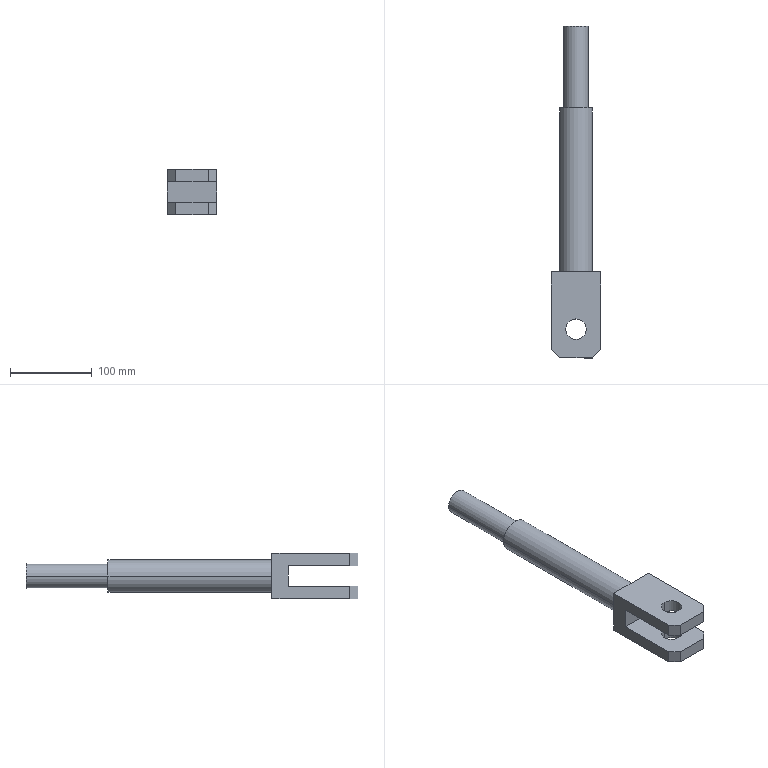Component | SolidWorks | Left-handTieRod1-1 | 1 solid | 24 faces | box 60 x 405 x 55 mm | volume 523287 mm3 | plane 16 | cylinder 8 | commonest cylinder face diameters 25 x4 30 x2 40 x2 | material N/A
build123d program:
from build123d import *

# Parameters (mm, degrees)
BOSS_EXTRUDE1_DEPTH = 30
SKETCH2_R           = 12.5
CUT_EXTRUDE1_DEPTH  = 60
CHAMFER1_SIZE       = 10
SKETCH3_R           = 20
BOSS_EXTRUDE2_DEPTH = 300
SKETCH4_OUTSIDE_W   = 144.62
SKETCH4_OUTSIDE_H   = 139.62
SKETCH4_OUTSIDE_R   = 15
CUT_EXTRUDE2_DEPTH  = 100


with BuildPart() as part:
    # Sketch1 → Boss-Extrude1 (new, symmetric)
    with BuildSketch(Plane(origin=(0, 0, 0), x_dir=(0, 0, -1), z_dir=(1, 0, 0))):
        Polygon((52.5, 12.5), (-32.5, 12.5), (-32.5, -12.5), (52.5, -12.5), (52.5, -27.5), (-52.5, -27.5), (-52.5, 27.5), (52.5, 27.5), align=None)
    extrude(amount=BOSS_EXTRUDE1_DEPTH, both=True)

    # Sketch2 → Cut-Extrude1 (cut)
    with BuildSketch(Plane.XZ.offset(27.5)):
        with Locations(Location((0, -17.5, 0), (0, 0, 270))):
            Circle(SKETCH2_R)
    extrude(amount=-CUT_EXTRUDE1_DEPTH, mode=Mode.SUBTRACT)

    # Chamfer1
    chamfer1_edges = [part.edges().sort_by_distance(p)[0] for p in [
        (-30, 20, -52.5),
        (30, -20, -52.5),
        (30, 20, -52.5),
        (-30, -20, -52.5),
    ]]
    chamfer(chamfer1_edges, length=CHAMFER1_SIZE)

    # Sketch3 → Boss-Extrude2 (add)
    with BuildSketch(Plane.XY.offset(52.5)):
        Circle(SKETCH3_R)
    extrude(amount=BOSS_EXTRUDE2_DEPTH)

    # Sketch4 outside → Cut-Extrude2 (cut)
    with BuildSketch(Plane.XY.offset(352.5)):
        Rectangle(SKETCH4_OUTSIDE_W, SKETCH4_OUTSIDE_H)
        Circle(SKETCH4_OUTSIDE_R, mode=Mode.SUBTRACT)
    extrude(amount=-CUT_EXTRUDE2_DEPTH, mode=Mode.SUBTRACT)


solid = part.part

# Placed as in the assembly
solid = solid.moved(Location((69.344, 70.287, 17), (-90, 0, 0)))
STEP:
#1=COLOUR_RGB('',0.7922,0.8196,0.9333);
#2=FILL_AREA_STYLE_COLOUR('',#1);
#3=FILL_AREA_STYLE('',(#2));
#4=SURFACE_STYLE_FILL_AREA(#3);
#5=SURFACE_SIDE_STYLE('',(#4));
#6=SURFACE_STYLE_USAGE(.BOTH.,#5);
#7=PRESENTATION_STYLE_ASSIGNMENT((#6));
#8=CARTESIAN_POINT('',(3.321,12.708,0.6693));
#9=VERTEX_POINT('',#8);
#10=CARTESIAN_POINT('',(2.14,12.708,0.6693));
#11=VERTEX_POINT('',#10);
#12=CARTESIAN_POINT('',(2.73,12.708,0.6693));
#13=DIRECTION('',(0.,1.,0.));
#14=DIRECTION('',(1.,-0.,0.));
#15=AXIS2_PLACEMENT_3D('',#12,#13,#14);
#16=CIRCLE('',#15,0.5906);
#17=EDGE_CURVE('',#9,#11,#16,.T.);
#18=ORIENTED_EDGE('',*,*,#17,.T.);
#19=CARTESIAN_POINT('',(2.14,16.645,0.6693));
#20=VERTEX_POINT('',#19);
#21=CARTESIAN_POINT('',(2.14,12.708,0.6693));
#22=DIRECTION('',(0.,1.,0.));
#23=VECTOR('',#22,39.37);
#24=LINE('',#21,#23);
#25=EDGE_CURVE('',#11,#20,#24,.T.);
#26=ORIENTED_EDGE('',*,*,#25,.T.);
#27=CARTESIAN_POINT('',(3.321,16.645,0.6693));
#28=VERTEX_POINT('',#27);
#29=CARTESIAN_POINT('',(2.73,16.645,0.6693));
#30=DIRECTION('',(0.,1.,0.));
#31=DIRECTION('',(1.,-0.,0.));
#32=AXIS2_PLACEMENT_3D('',#29,#30,#31);
#33=CIRCLE('',#32,0.5906);
#34=EDGE_CURVE('',#28,#20,#33,.T.);
#35=ORIENTED_EDGE('',*,*,#34,.F.);
#36=CARTESIAN_POINT('',(3.321,12.708,0.6693));
#37=DIRECTION('',(0.,1.,0.));
#38=VECTOR('',#37,39.37);
#39=LINE('',#36,#38);
#40=EDGE_CURVE('',#9,#28,#39,.T.);
#41=ORIENTED_EDGE('',*,*,#40,.F.);
#42=EDGE_LOOP('',(#18,#26,#35,#41));
#43=FACE_OUTER_BOUND('',#42,.T.);
#44=CARTESIAN_POINT('',(2.73,12.708,0.6693));
#45=DIRECTION('',(0.,1.,0.));
#46=DIRECTION('',(1.,-0.,0.));
#47=AXIS2_PLACEMENT_3D('',#44,#45,#46);
#48=CYLINDRICAL_SURFACE('',#47,0.5906);
#49=ADVANCED_FACE('',(#43),#48,.T.);
#50=CARTESIAN_POINT('',(2.73,2.57,1.161));
#51=VERTEX_POINT('',#50);
#52=CARTESIAN_POINT('',(2.73,1.586,1.161));
#53=VERTEX_POINT('',#52);
#54=CARTESIAN_POINT('',(2.73,2.078,1.161));
#55=DIRECTION('',(0.,-0.,1.));
#56=DIRECTION('',(-0.,-1.,0.));
#57=AXIS2_PLACEMENT_3D('',#54,#55,#56);
#58=CIRCLE('',#57,0.4921);
#59=EDGE_CURVE('',#51,#53,#58,.T.);
#60=ORIENTED_EDGE('',*,*,#59,.F.);
#61=CARTESIAN_POINT('',(2.73,2.57,1.752));
#62=VERTEX_POINT('',#61);
#63=CARTESIAN_POINT('',(2.73,2.57,-0.6102));
#64=DIRECTION('',(0.,-0.,1.));
#65=VECTOR('',#64,39.37);
#66=LINE('',#63,#65);
#67=EDGE_CURVE('',#51,#62,#66,.T.);
#68=ORIENTED_EDGE('',*,*,#67,.T.);
#69=CARTESIAN_POINT('',(2.73,1.586,1.752));
#70=VERTEX_POINT('',#69);
#71=CARTESIAN_POINT('',(2.73,2.078,1.752));
#72=DIRECTION('',(0.,-0.,1.));
#73=DIRECTION('',(-0.,-1.,-0.));
#74=AXIS2_PLACEMENT_3D('',#71,#72,#73);
#75=CIRCLE('',#74,0.4921);
#76=EDGE_CURVE('',#62,#70,#75,.T.);
#77=ORIENTED_EDGE('',*,*,#76,.T.);
#78=CARTESIAN_POINT('',(2.73,1.586,-0.6102));
#79=DIRECTION('',(0.,-0.,1.));
#80=VECTOR('',#79,39.37);
#81=LINE('',#78,#80);
#82=EDGE_CURVE('',#53,#70,#81,.T.);
#83=ORIENTED_EDGE('',*,*,#82,.F.);
#84=EDGE_LOOP('',(#60,#68,#77,#83));
#85=FACE_OUTER_BOUND('',#84,.T.);
#86=CARTESIAN_POINT('',(2.73,2.078,-0.6102));
#87=DIRECTION('',(0.,-0.,1.));
#88=DIRECTION('',(-0.,-1.,-0.));
#89=AXIS2_PLACEMENT_3D('',#86,#87,#88);
#90=CYLINDRICAL_SURFACE('',#89,0.4921);
#91=ADVANCED_FACE('',(#85),#90,.F.);
#92=CARTESIAN_POINT('',(2.73,2.57,-0.4134));
#93=VERTEX_POINT('',#92);
#94=CARTESIAN_POINT('',(2.73,1.586,-0.4134));
#95=VERTEX_POINT('',#94);
#96=CARTESIAN_POINT('',(2.73,2.078,-0.4134));
#97=DIRECTION('',(0.,-0.,1.));
#98=DIRECTION('',(-0.,-1.,-0.));
#99=AXIS2_PLACEMENT_3D('',#96,#97,#98);
#100=CIRCLE('',#99,0.4921);
#101=EDGE_CURVE('',#93,#95,#100,.T.);
#102=ORIENTED_EDGE('',*,*,#101,.F.);
#103=CARTESIAN_POINT('',(2.73,2.57,0.1772));
#104=VERTEX_POINT('',#103);
#105=CARTESIAN_POINT('',(2.73,2.57,-0.6102));
#106=DIRECTION('',(0.,-0.,1.));
#107=VECTOR('',#106,39.37);
#108=LINE('',#105,#107);
#109=EDGE_CURVE('',#93,#104,#108,.T.);
#110=ORIENTED_EDGE('',*,*,#109,.T.);
#111=CARTESIAN_POINT('',(2.73,1.586,0.1772));
#112=VERTEX_POINT('',#111);
#113=CARTESIAN_POINT('',(2.73,2.078,0.1772));
#114=DIRECTION('',(-0.,0.,-1.));
#115=DIRECTION('',(0.,1.,0.));
#116=AXIS2_PLACEMENT_3D('',#113,#114,#115);
#117=CIRCLE('',#116,0.4921);
#118=EDGE_CURVE('',#112,#104,#117,.T.);
#119=ORIENTED_EDGE('',*,*,#118,.F.);
#120=CARTESIAN_POINT('',(2.73,1.586,-0.6102));
#121=DIRECTION('',(0.,-0.,1.));
#122=VECTOR('',#121,39.37);
#123=LINE('',#120,#122);
#124=EDGE_CURVE('',#95,#112,#123,.T.);
#125=ORIENTED_EDGE('',*,*,#124,.F.);
#126=EDGE_LOOP('',(#102,#110,#119,#125));
#127=FACE_OUTER_BOUND('',#126,.T.);
#128=CARTESIAN_POINT('',(2.73,2.078,-0.6102));
#129=DIRECTION('',(0.,-0.,1.));
#130=DIRECTION('',(-0.,-1.,-0.));
#131=AXIS2_PLACEMENT_3D('',#128,#129,#130);
#132=CYLINDRICAL_SURFACE('',#131,0.4921);
#133=ADVANCED_FACE('',(#127),#132,.F.);
#134=CARTESIAN_POINT('',(3.517,12.708,0.6693));
#135=VERTEX_POINT('',#134);
#136=CARTESIAN_POINT('',(1.943,12.708,0.6693));
#137=VERTEX_POINT('',#136);
#138=CARTESIAN_POINT('',(2.73,12.708,0.6693));
#139=DIRECTION('',(0.,1.,0.));
#140=DIRECTION('',(1.,-0.,0.));
#141=AXIS2_PLACEMENT_3D('',#138,#139,#140);
#142=CIRCLE('',#141,0.7874);
#143=EDGE_CURVE('',#135,#137,#142,.T.);
#144=ORIENTED_EDGE('',*,*,#143,.F.);
#145=CARTESIAN_POINT('',(3.517,4.834,0.6693));
#146=VERTEX_POINT('',#145);
#147=CARTESIAN_POINT('',(3.517,16.645,0.6693));
#148=DIRECTION('',(-0.,-1.,-0.));
#149=VECTOR('',#148,39.37);
#150=LINE('',#147,#149);
#151=EDGE_CURVE('',#135,#146,#150,.T.);
#152=ORIENTED_EDGE('',*,*,#151,.T.);
#153=CARTESIAN_POINT('',(1.943,4.834,0.6693));
#154=VERTEX_POINT('',#153);
#155=CARTESIAN_POINT('',(2.73,4.834,0.6693));
#156=DIRECTION('',(0.,1.,0.));
#157=DIRECTION('',(1.,-0.,0.));
#158=AXIS2_PLACEMENT_3D('',#155,#156,#157);
#159=CIRCLE('',#158,0.7874);
#160=EDGE_CURVE('',#146,#154,#159,.T.);
#161=ORIENTED_EDGE('',*,*,#160,.T.);
#162=CARTESIAN_POINT('',(1.943,16.645,0.6693));
#163=DIRECTION('',(-0.,-1.,-0.));
#164=VECTOR('',#163,39.37);
#165=LINE('',#162,#164);
#166=EDGE_CURVE('',#137,#154,#165,.T.);
#167=ORIENTED_EDGE('',*,*,#166,.F.);
#168=EDGE_LOOP('',(#144,#152,#161,#167));
#169=FACE_OUTER_BOUND('',#168,.T.);
#170=CARTESIAN_POINT('',(2.73,16.645,0.6693));
#171=DIRECTION('',(-0.,-1.,-0.));
#172=DIRECTION('',(-1.,0.,0.));
#173=AXIS2_PLACEMENT_3D('',#170,#171,#172);
#174=CYLINDRICAL_SURFACE('',#173,0.7874);
#175=ADVANCED_FACE('',(#169),#174,.T.);
#176=ORIENTED_EDGE('',*,*,#151,.F.);
#177=CARTESIAN_POINT('',(2.73,12.708,0.6693));
#178=DIRECTION('',(0.,1.,0.));
#179=DIRECTION('',(1.,-0.,0.));
#180=AXIS2_PLACEMENT_3D('',#177,#178,#179);
#181=CIRCLE('',#180,0.7874);
#182=EDGE_CURVE('',#137,#135,#181,.T.);
#183=ORIENTED_EDGE('',*,*,#182,.F.);
#184=ORIENTED_EDGE('',*,*,#166,.T.);
#185=CARTESIAN_POINT('',(2.73,4.834,0.6693));
#186=DIRECTION('',(0.,1.,0.));
#187=DIRECTION('',(1.,-0.,0.));
#188=AXIS2_PLACEMENT_3D('',#185,#186,#187);
#189=CIRCLE('',#188,0.7874);
#190=EDGE_CURVE('',#154,#146,#189,.T.);
#191=ORIENTED_EDGE('',*,*,#190,.T.);
#192=EDGE_LOOP('',(#176,#183,#184,#191));
#193=FACE_OUTER_BOUND('',#192,.T.);
#194=CARTESIAN_POINT('',(2.73,16.645,0.6693));
#195=DIRECTION('',(-0.,-1.,-0.));
#196=DIRECTION('',(-1.,0.,0.));
#197=AXIS2_PLACEMENT_3D('',#194,#195,#196);
#198=CYLINDRICAL_SURFACE('',#197,0.7874);
#199=ADVANCED_FACE('',(#193),#198,.T.);
#200=CARTESIAN_POINT('',(3.517,0.7003,0.1772));
#201=VERTEX_POINT('',#200);
#202=CARTESIAN_POINT('',(1.943,0.7003,0.1772));
#203=VERTEX_POINT('',#202);
#204=CARTESIAN_POINT('',(3.911,0.7003,0.1772));
#205=DIRECTION('',(-1.,0.,0.));
#206=VECTOR('',#205,39.37);
#207=LINE('',#204,#206);
#208=EDGE_CURVE('',#201,#203,#207,.T.);
#209=ORIENTED_EDGE('',*,*,#208,.T.);
#210=CARTESIAN_POINT('',(1.943,0.7003,-0.4134));
#211=VERTEX_POINT('',#210);
#212=CARTESIAN_POINT('',(1.943,0.7003,-0.4134));
#213=DIRECTION('',(-0.,-0.,-1.));
#214=VECTOR('',#213,39.37);
#215=LINE('',#212,#214);
#216=EDGE_CURVE('',#203,#211,#215,.T.);
#217=ORIENTED_EDGE('',*,*,#216,.T.);
#218=CARTESIAN_POINT('',(3.517,0.7003,-0.4134));
#219=VERTEX_POINT('',#218);
#220=CARTESIAN_POINT('',(3.911,0.7003,-0.4134));
#221=DIRECTION('',(-1.,0.,0.));
#222=VECTOR('',#221,39.37);
#223=LINE('',#220,#222);
#224=EDGE_CURVE('',#219,#211,#223,.T.);
#225=ORIENTED_EDGE('',*,*,#224,.F.);
#226=CARTESIAN_POINT('',(3.517,0.7003,0.1772));
#227=DIRECTION('',(0.,0.,1.));
#228=VECTOR('',#227,39.37);
#229=LINE('',#226,#228);
#230=EDGE_CURVE('',#219,#201,#229,.T.);
#231=ORIENTED_EDGE('',*,*,#230,.T.);
#232=EDGE_LOOP('',(#209,#217,#225,#231));
#233=FACE_OUTER_BOUND('',#232,.T.);
#234=CARTESIAN_POINT('',(3.911,0.7003,0.1772));
#235=DIRECTION('',(0.,1.,-0.));
#236=DIRECTION('',(0.,0.,1.));
#237=AXIS2_PLACEMENT_3D('',#234,#235,#236);
#238=PLANE('',#237);
#239=ADVANCED_FACE('',(#233),#238,.F.);
#240=CARTESIAN_POINT('',(2.73,2.078,-0.4134));
#241=DIRECTION('',(0.,-0.,1.));
#242=DIRECTION('',(-0.,-1.,-0.));
#243=AXIS2_PLACEMENT_3D('',#240,#241,#242);
#244=CIRCLE('',#243,0.4921);
#245=EDGE_CURVE('',#95,#93,#244,.T.);
#246=ORIENTED_EDGE('',*,*,#245,.T.);
#247=ORIENTED_EDGE('',*,*,#101,.T.);
#248=EDGE_LOOP('',(#246,#247));
#249=FACE_BOUND('',#248,.T.);
#250=ORIENTED_EDGE('',*,*,#224,.T.);
#251=CARTESIAN_POINT('',(1.549,1.094,-0.4134));
#252=VERTEX_POINT('',#251);
#253=CARTESIAN_POINT('',(1.943,0.7003,-0.4134));
#254=DIRECTION('',(-0.7071,0.7071,0.));
#255=VECTOR('',#254,39.37);
#256=LINE('',#253,#255);
#257=EDGE_CURVE('',#211,#252,#256,.T.);
#258=ORIENTED_EDGE('',*,*,#257,.T.);
#259=CARTESIAN_POINT('',(1.549,4.834,-0.4134));
#260=VERTEX_POINT('',#259);
#261=CARTESIAN_POINT('',(1.549,4.834,-0.4134));
#262=DIRECTION('',(0.,1.,0.));
#263=VECTOR('',#262,39.37);
#264=LINE('',#261,#263);
#265=EDGE_CURVE('',#252,#260,#264,.T.);
#266=ORIENTED_EDGE('',*,*,#265,.T.);
#267=CARTESIAN_POINT('',(3.911,4.834,-0.4134));
#268=VERTEX_POINT('',#267);
#269=CARTESIAN_POINT('',(3.911,4.834,-0.4134));
#270=DIRECTION('',(-1.,0.,0.));
#271=VECTOR('',#270,39.37);
#272=LINE('',#269,#271);
#273=EDGE_CURVE('',#268,#260,#272,.T.);
#274=ORIENTED_EDGE('',*,*,#273,.F.);
#275=CARTESIAN_POINT('',(3.911,1.094,-0.4134));
#276=VERTEX_POINT('',#275);
#277=CARTESIAN_POINT('',(3.911,4.834,-0.4134));
#278=DIRECTION('',(0.,1.,0.));
#279=VECTOR('',#278,39.37);
#280=LINE('',#277,#279);
#281=EDGE_CURVE('',#276,#268,#280,.T.);
#282=ORIENTED_EDGE('',*,*,#281,.F.);
#283=CARTESIAN_POINT('',(3.911,1.094,-0.4134));
#284=DIRECTION('',(-0.7071,-0.7071,-0.));
#285=VECTOR('',#284,39.37);
#286=LINE('',#283,#285);
#287=EDGE_CURVE('',#276,#219,#286,.T.);
#288=ORIENTED_EDGE('',*,*,#287,.T.);
#289=EDGE_LOOP('',(#250,#258,#266,#274,#282,#288));
#290=FACE_OUTER_BOUND('',#289,.T.);
#291=CARTESIAN_POINT('',(3.911,4.834,-0.4134));
#292=DIRECTION('',(0.,-0.,1.));
#293=DIRECTION('',(-0.,-1.,-0.));
#294=AXIS2_PLACEMENT_3D('',#291,#292,#293);
#295=PLANE('',#294);
#296=ADVANCED_FACE('',(#249,#290),#295,.F.);
#297=ORIENTED_EDGE('',*,*,#190,.F.);
#298=ORIENTED_EDGE('',*,*,#160,.F.);
#299=EDGE_LOOP('',(#297,#298));
#300=FACE_BOUND('',#299,.T.);
#301=CARTESIAN_POINT('',(1.549,4.834,1.752));
#302=VERTEX_POINT('',#301);
#303=CARTESIAN_POINT('',(1.549,4.834,1.752));
#304=DIRECTION('',(0.,0.,1.));
#305=VECTOR('',#304,39.37);
#306=LINE('',#303,#305);
#307=EDGE_CURVE('',#260,#302,#306,.T.);
#308=ORIENTED_EDGE('',*,*,#307,.T.);
#309=CARTESIAN_POINT('',(3.911,4.834,1.752));
#310=VERTEX_POINT('',#309);
#311=CARTESIAN_POINT('',(3.911,4.834,1.752));
#312=DIRECTION('',(-1.,0.,0.));
#313=VECTOR('',#312,39.37);
#314=LINE('',#311,#313);
#315=EDGE_CURVE('',#310,#302,#314,.T.);
#316=ORIENTED_EDGE('',*,*,#315,.F.);
#317=CARTESIAN_POINT('',(3.911,4.834,1.752));
#318=DIRECTION('',(0.,0.,1.));
#319=VECTOR('',#318,39.37);
#320=LINE('',#317,#319);
#321=EDGE_CURVE('',#268,#310,#320,.T.);
#322=ORIENTED_EDGE('',*,*,#321,.F.);
#323=ORIENTED_EDGE('',*,*,#273,.T.);
#324=EDGE_LOOP('',(#308,#316,#322,#323));
#325=FACE_OUTER_BOUND('',#324,.T.);
#326=CARTESIAN_POINT('',(3.911,4.834,1.752));
#327=DIRECTION('',(-0.,-1.,0.));
#328=DIRECTION('',(-0.,-0.,-1.));
#329=AXIS2_PLACEMENT_3D('',#326,#327,#328);
#330=PLANE('',#329);
#331=ADVANCED_FACE('',(#300,#325),#330,.F.);
#332=CARTESIAN_POINT('',(2.73,2.078,1.752));
#333=DIRECTION('',(0.,-0.,1.));
#334=DIRECTION('',(-0.,-1.,-0.));
#335=AXIS2_PLACEMENT_3D('',#332,#333,#334);
#336=CIRCLE('',#335,0.4921);
#337=EDGE_CURVE('',#70,#62,#336,.T.);
#338=ORIENTED_EDGE('',*,*,#337,.F.);
#339=ORIENTED_EDGE('',*,*,#76,.F.);
#340=EDGE_LOOP('',(#338,#339));
#341=FACE_BOUND('',#340,.T.);
#342=CARTESIAN_POINT('',(1.549,1.094,1.752));
#343=VERTEX_POINT('',#342);
#344=CARTESIAN_POINT('',(1.549,4.834,1.752));
#345=DIRECTION('',(-0.,-1.,0.));
#346=VECTOR('',#345,39.37);
#347=LINE('',#344,#346);
#348=EDGE_CURVE('',#302,#343,#347,.T.);
#349=ORIENTED_EDGE('',*,*,#348,.T.);
#350=CARTESIAN_POINT('',(1.943,0.7003,1.752));
#351=VERTEX_POINT('',#350);
#352=CARTESIAN_POINT('',(1.943,0.7003,1.752));
#353=DIRECTION('',(0.7071,-0.7071,0.));
#354=VECTOR('',#353,39.37);
#355=LINE('',#352,#354);
#356=EDGE_CURVE('',#343,#351,#355,.T.);
#357=ORIENTED_EDGE('',*,*,#356,.T.);
#358=CARTESIAN_POINT('',(3.517,0.7003,1.752));
#359=VERTEX_POINT('',#358);
#360=CARTESIAN_POINT('',(3.911,0.7003,1.752));
#361=DIRECTION('',(-1.,0.,0.));
#362=VECTOR('',#361,39.37);
#363=LINE('',#360,#362);
#364=EDGE_CURVE('',#359,#351,#363,.T.);
#365=ORIENTED_EDGE('',*,*,#364,.F.);
#366=CARTESIAN_POINT('',(3.911,1.094,1.752));
#367=VERTEX_POINT('',#366);
#368=CARTESIAN_POINT('',(3.911,1.094,1.752));
#369=DIRECTION('',(0.7071,0.7071,-0.));
#370=VECTOR('',#369,39.37);
#371=LINE('',#368,#370);
#372=EDGE_CURVE('',#359,#367,#371,.T.);
#373=ORIENTED_EDGE('',*,*,#372,.T.);
#374=CARTESIAN_POINT('',(3.911,4.834,1.752));
#375=DIRECTION('',(-0.,-1.,0.));
#376=VECTOR('',#375,39.37);
#377=LINE('',#374,#376);
#378=EDGE_CURVE('',#310,#367,#377,.T.);
#379=ORIENTED_EDGE('',*,*,#378,.F.);
#380=ORIENTED_EDGE('',*,*,#315,.T.);
#381=EDGE_LOOP('',(#349,#357,#365,#373,#379,#380));
#382=FACE_OUTER_BOUND('',#381,.T.);
#383=CARTESIAN_POINT('',(3.911,4.834,1.752));
#384=DIRECTION('',(-0.,-0.,-1.));
#385=DIRECTION('',(0.,1.,-0.));
#386=AXIS2_PLACEMENT_3D('',#383,#384,#385);
#387=PLANE('',#386);
#388=ADVANCED_FACE('',(#341,#382),#387,.F.);
#389=ORIENTED_EDGE('',*,*,#364,.T.);
#390=CARTESIAN_POINT('',(1.943,0.7003,1.161));
#391=VERTEX_POINT('',#390);
#392=CARTESIAN_POINT('',(1.943,0.7003,1.161));
#393=DIRECTION('',(-0.,0.,-1.));
#394=VECTOR('',#393,39.37);
#395=LINE('',#392,#394);
#396=EDGE_CURVE('',#351,#391,#395,.T.);
#397=ORIENTED_EDGE('',*,*,#396,.T.);
#398=CARTESIAN_POINT('',(3.517,0.7003,1.161));
#399=VERTEX_POINT('',#398);
#400=CARTESIAN_POINT('',(3.911,0.7003,1.161));
#401=DIRECTION('',(-1.,0.,0.));
#402=VECTOR('',#401,39.37);
#403=LINE('',#400,#402);
#404=EDGE_CURVE('',#399,#391,#403,.T.);
#405=ORIENTED_EDGE('',*,*,#404,.F.);
#406=CARTESIAN_POINT('',(3.517,0.7003,1.752));
#407=DIRECTION('',(0.,-0.,1.));
#408=VECTOR('',#407,39.37);
#409=LINE('',#406,#408);
#410=EDGE_CURVE('',#399,#359,#409,.T.);
#411=ORIENTED_EDGE('',*,*,#410,.T.);
#412=EDGE_LOOP('',(#389,#397,#405,#411));
#413=FACE_OUTER_BOUND('',#412,.T.);
#414=CARTESIAN_POINT('',(3.911,0.7003,1.752));
#415=DIRECTION('',(0.,1.,0.));
#416=DIRECTION('',(0.,-0.,1.));
#417=AXIS2_PLACEMENT_3D('',#414,#415,#416);
#418=PLANE('',#417);
#419=ADVANCED_FACE('',(#413),#418,.F.);
#420=CARTESIAN_POINT('',(2.73,2.078,1.161));
#421=DIRECTION('',(0.,-0.,1.));
#422=DIRECTION('',(-0.,-1.,0.));
#423=AXIS2_PLACEMENT_3D('',#420,#421,#422);
#424=CIRCLE('',#423,0.4921);
#425=EDGE_CURVE('',#53,#51,#424,.T.);
#426=ORIENTED_EDGE('',*,*,#425,.T.);
#427=ORIENTED_EDGE('',*,*,#59,.T.);
#428=EDGE_LOOP('',(#426,#427));
#429=FACE_BOUND('',#428,.T.);
#430=ORIENTED_EDGE('',*,*,#404,.T.);
#431=CARTESIAN_POINT('',(1.549,1.094,1.161));
#432=VERTEX_POINT('',#431);
#433=CARTESIAN_POINT('',(1.943,0.7003,1.161));
#434=DIRECTION('',(-0.7071,0.7071,0.));
#435=VECTOR('',#434,39.37);
#436=LINE('',#433,#435);
#437=EDGE_CURVE('',#391,#432,#436,.T.);
#438=ORIENTED_EDGE('',*,*,#437,.T.);
#439=CARTESIAN_POINT('',(1.549,4.047,1.161));
#440=VERTEX_POINT('',#439);
#441=CARTESIAN_POINT('',(1.549,4.047,1.161));
#442=DIRECTION('',(0.,1.,0.));
#443=VECTOR('',#442,39.37);
#444=LINE('',#441,#443);
#445=EDGE_CURVE('',#432,#440,#444,.T.);
#446=ORIENTED_EDGE('',*,*,#445,.T.);
#447=CARTESIAN_POINT('',(3.911,4.047,1.161));
#448=VERTEX_POINT('',#447);
#449=CARTESIAN_POINT('',(3.911,4.047,1.161));
#450=DIRECTION('',(-1.,0.,0.));
#451=VECTOR('',#450,39.37);
#452=LINE('',#449,#451);
#453=EDGE_CURVE('',#448,#440,#452,.T.);
#454=ORIENTED_EDGE('',*,*,#453,.F.);
#455=CARTESIAN_POINT('',(3.911,1.094,1.161));
#456=VERTEX_POINT('',#455);
#457=CARTESIAN_POINT('',(3.911,4.047,1.161));
#458=DIRECTION('',(0.,1.,0.));
#459=VECTOR('',#458,39.37);
#460=LINE('',#457,#459);
#461=EDGE_CURVE('',#456,#448,#460,.T.);
#462=ORIENTED_EDGE('',*,*,#461,.F.);
#463=CARTESIAN_POINT('',(3.911,1.094,1.161));
#464=DIRECTION('',(-0.7071,-0.7071,-0.));
#465=VECTOR('',#464,39.37);
#466=LINE('',#463,#465);
#467=EDGE_CURVE('',#456,#399,#466,.T.);
#468=ORIENTED_EDGE('',*,*,#467,.T.);
#469=EDGE_LOOP('',(#430,#438,#446,#454,#462,#468));
#470=FACE_OUTER_BOUND('',#469,.T.);
#471=CARTESIAN_POINT('',(3.911,4.047,1.161));
#472=DIRECTION('',(0.,-0.,1.));
#473=DIRECTION('',(-0.,-1.,-0.));
#474=AXIS2_PLACEMENT_3D('',#471,#472,#473);
#475=PLANE('',#474);
#476=ADVANCED_FACE('',(#429,#470),#475,.F.);
#477=CARTESIAN_POINT('',(1.549,4.047,0.1772));
#478=VERTEX_POINT('',#477);
#479=CARTESIAN_POINT('',(1.549,4.047,0.1772));
#480=DIRECTION('',(-0.,0.,-1.));
#481=VECTOR('',#480,39.37);
#482=LINE('',#479,#481);
#483=EDGE_CURVE('',#440,#478,#482,.T.);
#484=ORIENTED_EDGE('',*,*,#483,.T.);
#485=CARTESIAN_POINT('',(3.911,4.047,0.1772));
#486=VERTEX_POINT('',#485);
#487=CARTESIAN_POINT('',(3.911,4.047,0.1772));
#488=DIRECTION('',(-1.,0.,0.));
#489=VECTOR('',#488,39.37);
#490=LINE('',#487,#489);
#491=EDGE_CURVE('',#486,#478,#490,.T.);
#492=ORIENTED_EDGE('',*,*,#491,.F.);
#493=CARTESIAN_POINT('',(3.911,4.047,0.1772));
#494=DIRECTION('',(-0.,0.,-1.));
#495=VECTOR('',#494,39.37);
#496=LINE('',#493,#495);
#497=EDGE_CURVE('',#448,#486,#496,.T.);
#498=ORIENTED_EDGE('',*,*,#497,.F.);
#499=ORIENTED_EDGE('',*,*,#453,.T.);
#500=EDGE_LOOP('',(#484,#492,#498,#499));
#501=FACE_OUTER_BOUND('',#500,.T.);
#502=CARTESIAN_POINT('',(3.911,4.047,0.1772));
#503=DIRECTION('',(0.,1.,0.));
#504=DIRECTION('',(1.,-0.,-0.));
#505=AXIS2_PLACEMENT_3D('',#502,#503,#504);
#506=PLANE('',#505);
#507=ADVANCED_FACE('',(#501),#506,.F.);
#508=ORIENTED_EDGE('',*,*,#118,.T.);
#509=CARTESIAN_POINT('',(2.73,2.078,0.1772));
#510=DIRECTION('',(-0.,0.,-1.));
#511=DIRECTION('',(0.,1.,0.));
#512=AXIS2_PLACEMENT_3D('',#509,#510,#511);
#513=CIRCLE('',#512,0.4921);
#514=EDGE_CURVE('',#104,#112,#513,.T.);
#515=ORIENTED_EDGE('',*,*,#514,.T.);
#516=EDGE_LOOP('',(#508,#515));
#517=FACE_BOUND('',#516,.T.);
#518=CARTESIAN_POINT('',(1.549,1.094,0.1772));
#519=VERTEX_POINT('',#518);
#520=CARTESIAN_POINT('',(1.549,0.7003,0.1772));
#521=DIRECTION('',(-0.,-1.,-0.));
#522=VECTOR('',#521,39.37);
#523=LINE('',#520,#522);
#524=EDGE_CURVE('',#478,#519,#523,.T.);
#525=ORIENTED_EDGE('',*,*,#524,.T.);
#526=CARTESIAN_POINT('',(1.943,0.7003,0.1772));
#527=DIRECTION('',(0.7071,-0.7071,-0.));
#528=VECTOR('',#527,39.37);
#529=LINE('',#526,#528);
#530=EDGE_CURVE('',#519,#203,#529,.T.);
#531=ORIENTED_EDGE('',*,*,#530,.T.);
#532=ORIENTED_EDGE('',*,*,#208,.F.);
#533=CARTESIAN_POINT('',(3.911,1.094,0.1772));
#534=VERTEX_POINT('',#533);
#535=CARTESIAN_POINT('',(3.911,1.094,0.1772));
#536=DIRECTION('',(0.7071,0.7071,0.));
#537=VECTOR('',#536,39.37);
#538=LINE('',#535,#537);
#539=EDGE_CURVE('',#201,#534,#538,.T.);
#540=ORIENTED_EDGE('',*,*,#539,.T.);
#541=CARTESIAN_POINT('',(3.911,0.7003,0.1772));
#542=DIRECTION('',(-0.,-1.,-0.));
#543=VECTOR('',#542,39.37);
#544=LINE('',#541,#543);
#545=EDGE_CURVE('',#486,#534,#544,.T.);
#546=ORIENTED_EDGE('',*,*,#545,.F.);
#547=ORIENTED_EDGE('',*,*,#491,.T.);
#548=EDGE_LOOP('',(#525,#531,#532,#540,#546,#547));
#549=FACE_OUTER_BOUND('',#548,.T.);
#550=CARTESIAN_POINT('',(3.911,0.7003,0.1772));
#551=DIRECTION('',(-0.,0.,-1.));
#552=DIRECTION('',(0.,1.,0.));
#553=AXIS2_PLACEMENT_3D('',#550,#551,#552);
#554=PLANE('',#553);
#555=ADVANCED_FACE('',(#517,#549),#554,.F.);
#556=ORIENTED_EDGE('',*,*,#545,.T.);
#557=CARTESIAN_POINT('',(3.911,1.094,0.6693));
#558=DIRECTION('',(-0.,-0.,-1.));
#559=VECTOR('',#558,39.37);
#560=LINE('',#557,#559);
#561=EDGE_CURVE('',#534,#276,#560,.T.);
#562=ORIENTED_EDGE('',*,*,#561,.T.);
#563=ORIENTED_EDGE('',*,*,#281,.T.);
#564=ORIENTED_EDGE('',*,*,#321,.T.);
#565=ORIENTED_EDGE('',*,*,#378,.T.);
#566=CARTESIAN_POINT('',(3.911,1.094,0.6693));
#567=DIRECTION('',(-0.,0.,-1.));
#568=VECTOR('',#567,39.37);
#569=LINE('',#566,#568);
#570=EDGE_CURVE('',#367,#456,#569,.T.);
#571=ORIENTED_EDGE('',*,*,#570,.T.);
#572=ORIENTED_EDGE('',*,*,#461,.T.);
#573=ORIENTED_EDGE('',*,*,#497,.T.);
#574=EDGE_LOOP('',(#556,#562,#563,#564,#565,#571,#572,#573));
#575=FACE_OUTER_BOUND('',#574,.T.);
#576=CARTESIAN_POINT('',(3.911,2.767,0.6693));
#577=DIRECTION('',(-1.,0.,0.));
#578=DIRECTION('',(0.,1.,0.));
#579=AXIS2_PLACEMENT_3D('',#576,#577,#578);
#580=PLANE('',#579);
#581=ADVANCED_FACE('',(#575),#580,.F.);
#582=ORIENTED_EDGE('',*,*,#265,.F.);
#583=CARTESIAN_POINT('',(1.549,1.094,0.1772));
#584=DIRECTION('',(0.,0.,1.));
#585=VECTOR('',#584,39.37);
#586=LINE('',#583,#585);
#587=EDGE_CURVE('',#252,#519,#586,.T.);
#588=ORIENTED_EDGE('',*,*,#587,.T.);
#589=ORIENTED_EDGE('',*,*,#524,.F.);
#590=ORIENTED_EDGE('',*,*,#483,.F.);
#591=ORIENTED_EDGE('',*,*,#445,.F.);
#592=CARTESIAN_POINT('',(1.549,1.094,1.752));
#593=DIRECTION('',(0.,-0.,1.));
#594=VECTOR('',#593,39.37);
#595=LINE('',#592,#594);
#596=EDGE_CURVE('',#432,#343,#595,.T.);
#597=ORIENTED_EDGE('',*,*,#596,.T.);
#598=ORIENTED_EDGE('',*,*,#348,.F.);
#599=ORIENTED_EDGE('',*,*,#307,.F.);
#600=EDGE_LOOP('',(#582,#588,#589,#590,#591,#597,#598,#599));
#601=FACE_OUTER_BOUND('',#600,.T.);
#602=CARTESIAN_POINT('',(1.549,2.767,0.6693));
#603=DIRECTION('',(-1.,0.,0.));
#604=DIRECTION('',(0.,1.,0.));
#605=AXIS2_PLACEMENT_3D('',#602,#603,#604);
#606=PLANE('',#605);
#607=ADVANCED_FACE('',(#601),#606,.T.);
#608=ORIENTED_EDGE('',*,*,#109,.F.);
#609=ORIENTED_EDGE('',*,*,#245,.F.);
#610=ORIENTED_EDGE('',*,*,#124,.T.);
#611=ORIENTED_EDGE('',*,*,#514,.F.);
#612=EDGE_LOOP('',(#608,#609,#610,#611));
#613=FACE_OUTER_BOUND('',#612,.T.);
#614=CARTESIAN_POINT('',(2.73,2.078,-0.6102));
#615=DIRECTION('',(0.,-0.,1.));
#616=DIRECTION('',(-0.,-1.,-0.));
#617=AXIS2_PLACEMENT_3D('',#614,#615,#616);
#618=CYLINDRICAL_SURFACE('',#617,0.4921);
#619=ADVANCED_FACE('',(#613),#618,.F.);
#620=ORIENTED_EDGE('',*,*,#67,.F.);
#621=ORIENTED_EDGE('',*,*,#425,.F.);
#622=ORIENTED_EDGE('',*,*,#82,.T.);
#623=ORIENTED_EDGE('',*,*,#337,.T.);
#624=EDGE_LOOP('',(#620,#621,#622,#623));
#625=FACE_OUTER_BOUND('',#624,.T.);
#626=CARTESIAN_POINT('',(2.73,2.078,-0.6102));
#627=DIRECTION('',(0.,-0.,1.));
#628=DIRECTION('',(-0.,-1.,-0.));
#629=AXIS2_PLACEMENT_3D('',#626,#627,#628);
#630=CYLINDRICAL_SURFACE('',#629,0.4921);
#631=ADVANCED_FACE('',(#625),#630,.F.);
#632=ORIENTED_EDGE('',*,*,#530,.F.);
#633=ORIENTED_EDGE('',*,*,#587,.F.);
#634=ORIENTED_EDGE('',*,*,#257,.F.);
#635=ORIENTED_EDGE('',*,*,#216,.F.);
#636=EDGE_LOOP('',(#632,#633,#634,#635));
#637=FACE_OUTER_BOUND('',#636,.T.);
#638=CARTESIAN_POINT('',(1.943,0.7003,0.1772));
#639=DIRECTION('',(-0.7071,-0.7071,0.));
#640=DIRECTION('',(0.,0.,1.));
#641=AXIS2_PLACEMENT_3D('',#638,#639,#640);
#642=PLANE('',#641);
#643=ADVANCED_FACE('',(#637),#642,.T.);
#644=ORIENTED_EDGE('',*,*,#356,.F.);
#645=ORIENTED_EDGE('',*,*,#596,.F.);
#646=ORIENTED_EDGE('',*,*,#437,.F.);
#647=ORIENTED_EDGE('',*,*,#396,.F.);
#648=EDGE_LOOP('',(#644,#645,#646,#647));
#649=FACE_OUTER_BOUND('',#648,.T.);
#650=CARTESIAN_POINT('',(1.943,0.7003,1.752));
#651=DIRECTION('',(-0.7071,-0.7071,-0.));
#652=DIRECTION('',(0.,-0.,1.));
#653=AXIS2_PLACEMENT_3D('',#650,#651,#652);
#654=PLANE('',#653);
#655=ADVANCED_FACE('',(#649),#654,.T.);
#656=ORIENTED_EDGE('',*,*,#539,.F.);
#657=ORIENTED_EDGE('',*,*,#230,.F.);
#658=ORIENTED_EDGE('',*,*,#287,.F.);
#659=ORIENTED_EDGE('',*,*,#561,.F.);
#660=EDGE_LOOP('',(#656,#657,#658,#659));
#661=FACE_OUTER_BOUND('',#660,.T.);
#662=CARTESIAN_POINT('',(3.911,1.094,0.6693));
#663=DIRECTION('',(-0.7071,0.7071,-0.));
#664=DIRECTION('',(-0.,-0.,-1.));
#665=AXIS2_PLACEMENT_3D('',#662,#663,#664);
#666=PLANE('',#665);
#667=ADVANCED_FACE('',(#661),#666,.F.);
#668=ORIENTED_EDGE('',*,*,#372,.F.);
#669=ORIENTED_EDGE('',*,*,#410,.F.);
#670=ORIENTED_EDGE('',*,*,#467,.F.);
#671=ORIENTED_EDGE('',*,*,#570,.F.);
#672=EDGE_LOOP('',(#668,#669,#670,#671));
#673=FACE_OUTER_BOUND('',#672,.T.);
#674=CARTESIAN_POINT('',(3.911,1.094,0.6693));
#675=DIRECTION('',(-0.7071,0.7071,0.));
#676=DIRECTION('',(-0.,0.,-1.));
#677=AXIS2_PLACEMENT_3D('',#674,#675,#676);
#678=PLANE('',#677);
#679=ADVANCED_FACE('',(#673),#678,.F.);
#680=ORIENTED_EDGE('',*,*,#17,.F.);
#681=CARTESIAN_POINT('',(2.73,12.708,0.6693));
#682=DIRECTION('',(0.,1.,0.));
#683=DIRECTION('',(1.,-0.,0.));
#684=AXIS2_PLACEMENT_3D('',#681,#682,#683);
#685=CIRCLE('',#684,0.5906);
#686=EDGE_CURVE('',#11,#9,#685,.T.);
#687=ORIENTED_EDGE('',*,*,#686,.F.);
#688=EDGE_LOOP('',(#680,#687));
#689=FACE_BOUND('',#688,.T.);
#690=ORIENTED_EDGE('',*,*,#182,.T.);
#691=ORIENTED_EDGE('',*,*,#143,.T.);
#692=EDGE_LOOP('',(#690,#691));
#693=FACE_OUTER_BOUND('',#692,.T.);
#694=CARTESIAN_POINT('',(2.73,12.708,0.6693));
#695=DIRECTION('',(0.,1.,0.));
#696=DIRECTION('',(1.,-0.,-0.));
#697=AXIS2_PLACEMENT_3D('',#694,#695,#696);
#698=PLANE('',#697);
#699=ADVANCED_FACE('',(#689,#693),#698,.T.);
#700=ORIENTED_EDGE('',*,*,#25,.F.);
#701=ORIENTED_EDGE('',*,*,#686,.T.);
#702=ORIENTED_EDGE('',*,*,#40,.T.);
#703=CARTESIAN_POINT('',(2.73,16.645,0.6693));
#704=DIRECTION('',(0.,1.,0.));
#705=DIRECTION('',(1.,-0.,0.));
#706=AXIS2_PLACEMENT_3D('',#703,#704,#705);
#707=CIRCLE('',#706,0.5906);
#708=EDGE_CURVE('',#20,#28,#707,.T.);
#709=ORIENTED_EDGE('',*,*,#708,.F.);
#710=EDGE_LOOP('',(#700,#701,#702,#709));
#711=FACE_OUTER_BOUND('',#710,.T.);
#712=CARTESIAN_POINT('',(2.73,12.708,0.6693));
#713=DIRECTION('',(0.,1.,0.));
#714=DIRECTION('',(1.,-0.,0.));
#715=AXIS2_PLACEMENT_3D('',#712,#713,#714);
#716=CYLINDRICAL_SURFACE('',#715,0.5906);
#717=ADVANCED_FACE('',(#711),#716,.T.);
#718=ORIENTED_EDGE('',*,*,#34,.T.);
#719=ORIENTED_EDGE('',*,*,#708,.T.);
#720=EDGE_LOOP('',(#718,#719));
#721=FACE_OUTER_BOUND('',#720,.T.);
#722=CARTESIAN_POINT('',(2.73,16.645,0.6693));
#723=DIRECTION('',(0.,1.,0.));
#724=DIRECTION('',(1.,-0.,-0.));
#725=AXIS2_PLACEMENT_3D('',#722,#723,#724);
#726=PLANE('',#725);
#727=ADVANCED_FACE('',(#721),#726,.T.);
#728=CLOSED_SHELL('',(#49,#91,#133,#175,#199,#239,#296,#331,#388,#419,#476,#507,#555,#581,#607,#619,#631,#643,#655,#667,#679,#699,#717,#727));
#729=MANIFOLD_SOLID_BREP('',#728);
#730=STYLED_ITEM('',(#7),#729);
#731=PRESENTATION_LAYER_ASSIGNMENT('','',(#730));
#732=(LENGTH_UNIT()NAMED_UNIT(*)SI_UNIT($,.METRE.));
#733=LENGTH_MEASURE_WITH_UNIT(LENGTH_MEASURE(0.0254),#732);
#734=DIMENSIONAL_EXPONENTS(1.,0.,0.,0.,0.,0.,0.);
#735=(CONVERSION_BASED_UNIT('',#733)LENGTH_UNIT()NAMED_UNIT(#734));
#736=UNCERTAINTY_MEASURE_WITH_UNIT(LENGTH_MEASURE(0.00001),#735,'','');
#737=(NAMED_UNIT(*)PLANE_ANGLE_UNIT()SI_UNIT($,.RADIAN.));
#738=(NAMED_UNIT(*)SI_UNIT($,.STERADIAN.)SOLID_ANGLE_UNIT());
#739=(GEOMETRIC_REPRESENTATION_CONTEXT(3)GLOBAL_UNCERTAINTY_ASSIGNED_CONTEXT((#736))GLOBAL_UNIT_ASSIGNED_CONTEXT((#735,#737,#738))REPRESENTATION_CONTEXT('',''));
#740=MECHANICAL_DESIGN_GEOMETRIC_PRESENTATION_REPRESENTATION('',(#730),#739);
#741=CARTESIAN_POINT('',(0.,0.,0.));
#742=DIRECTION('',(0.,0.,1.));
#743=DIRECTION('',(1.,0.,0.));
#744=AXIS2_PLACEMENT_3D('',#741,#742,#743);
#745=(LENGTH_UNIT()NAMED_UNIT(*)SI_UNIT($,.METRE.));
#746=LENGTH_MEASURE_WITH_UNIT(LENGTH_MEASURE(0.0254),#745);
#747=DIMENSIONAL_EXPONENTS(1.,0.,0.,0.,0.,0.,0.);
#748=(CONVERSION_BASED_UNIT('',#746)LENGTH_UNIT()NAMED_UNIT(#747));
#749=UNCERTAINTY_MEASURE_WITH_UNIT(LENGTH_MEASURE(0.00001),#748,'','');
#750=(NAMED_UNIT(*)PLANE_ANGLE_UNIT()SI_UNIT($,.RADIAN.));
#751=(NAMED_UNIT(*)SI_UNIT($,.STERADIAN.)SOLID_ANGLE_UNIT());
#752=(GEOMETRIC_REPRESENTATION_CONTEXT(3)GLOBAL_UNCERTAINTY_ASSIGNED_CONTEXT((#749))GLOBAL_UNIT_ASSIGNED_CONTEXT((#748,#750,#751))REPRESENTATION_CONTEXT('',''));
#753=ADVANCED_BREP_SHAPE_REPRESENTATION('',(#729,#744),#752);